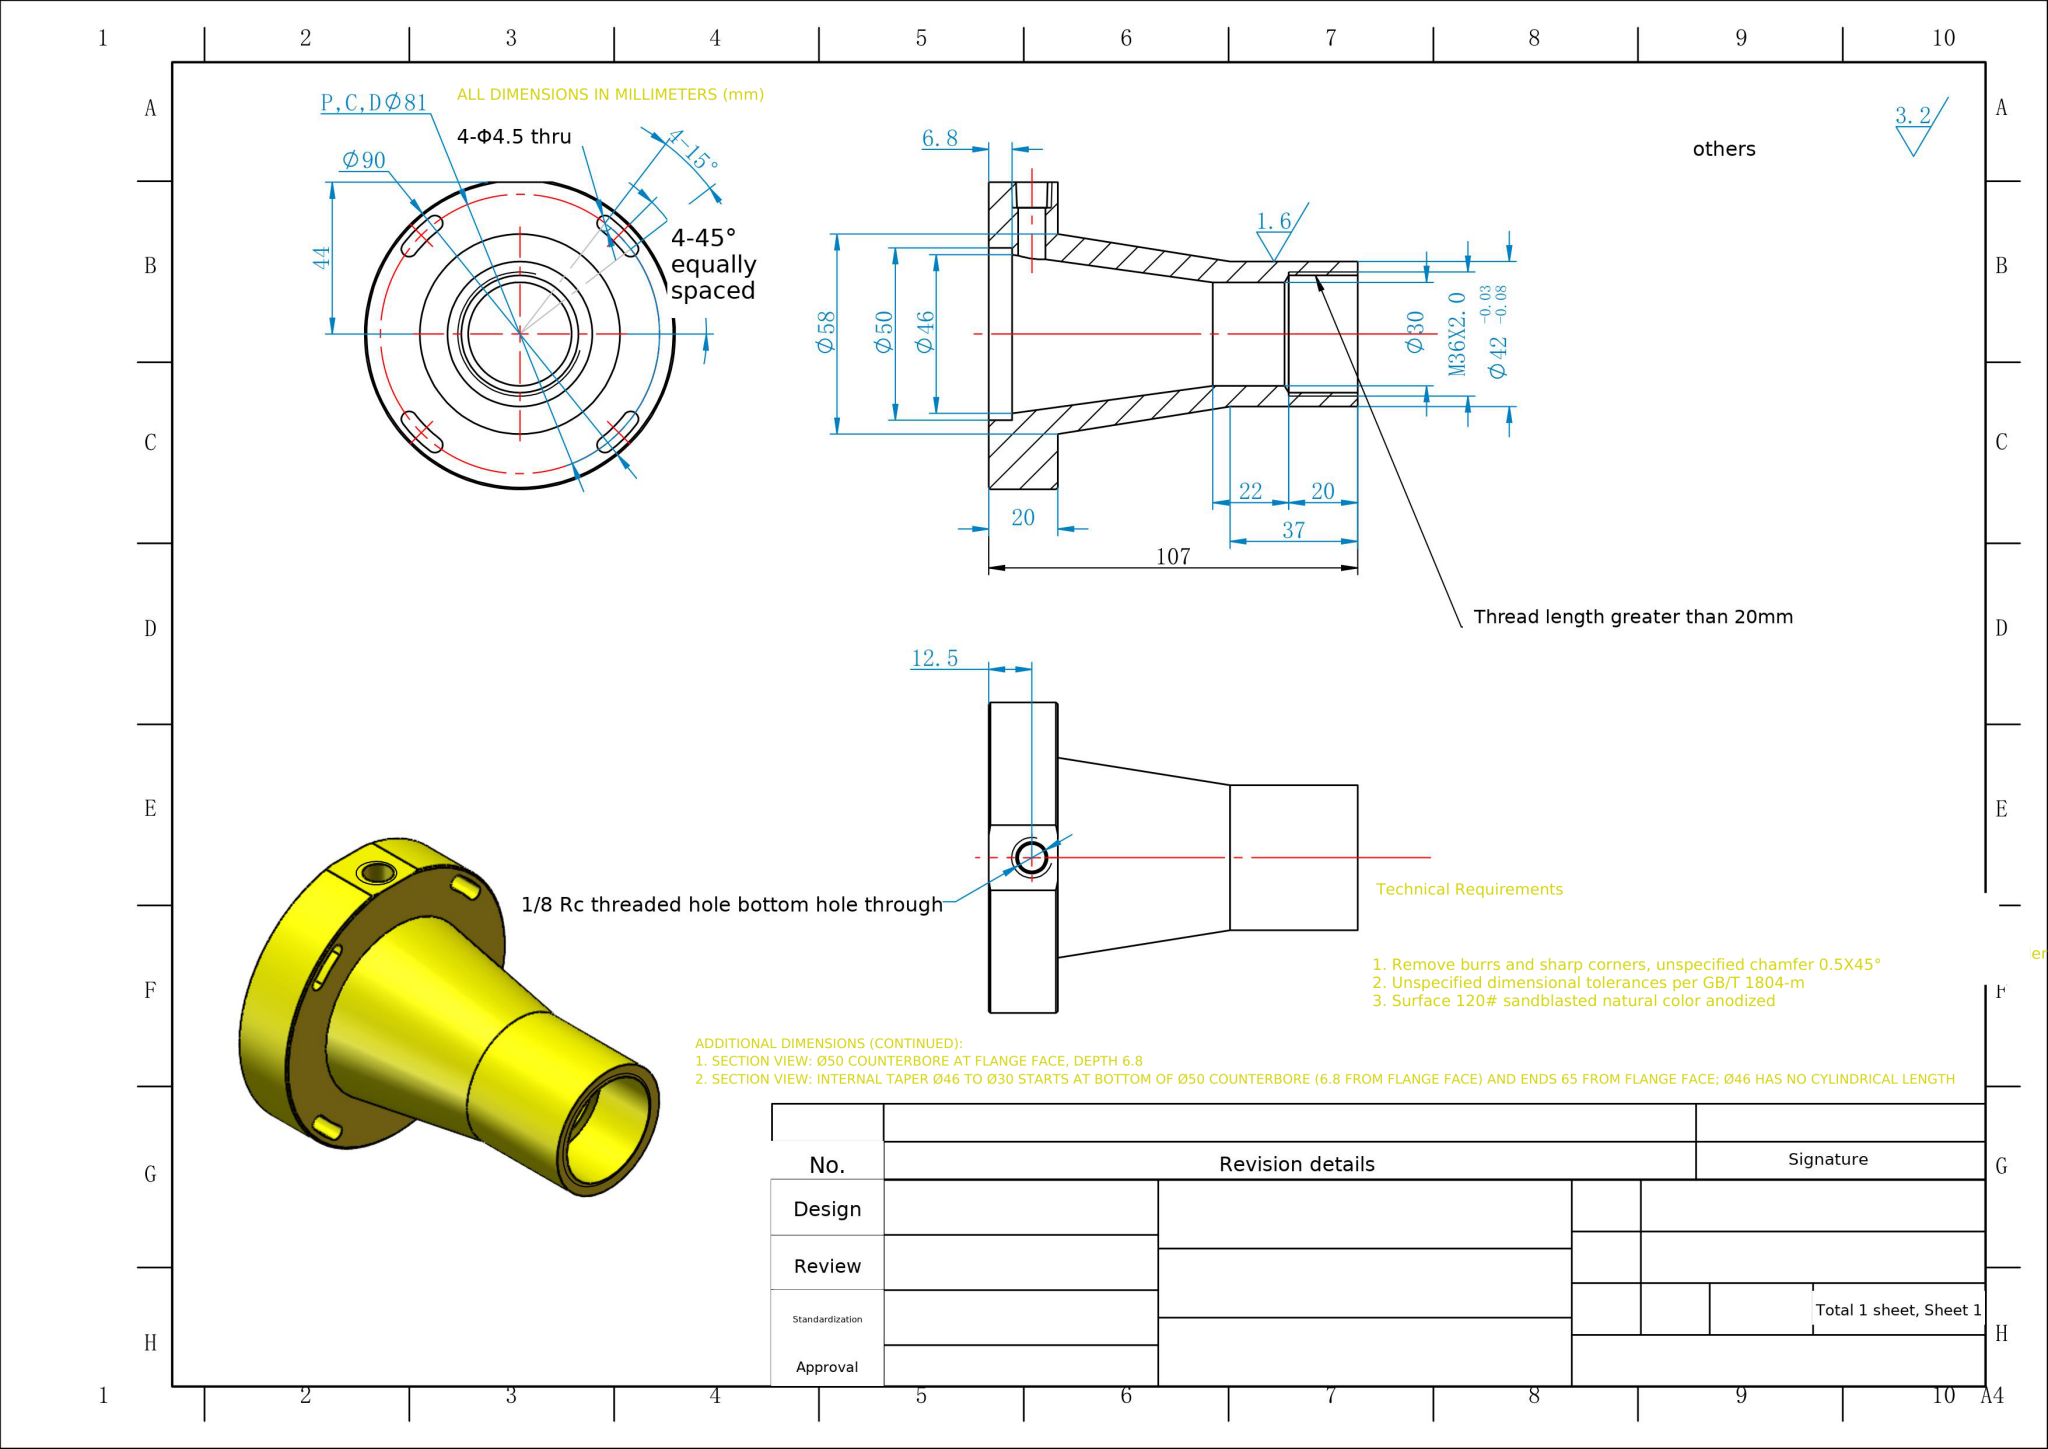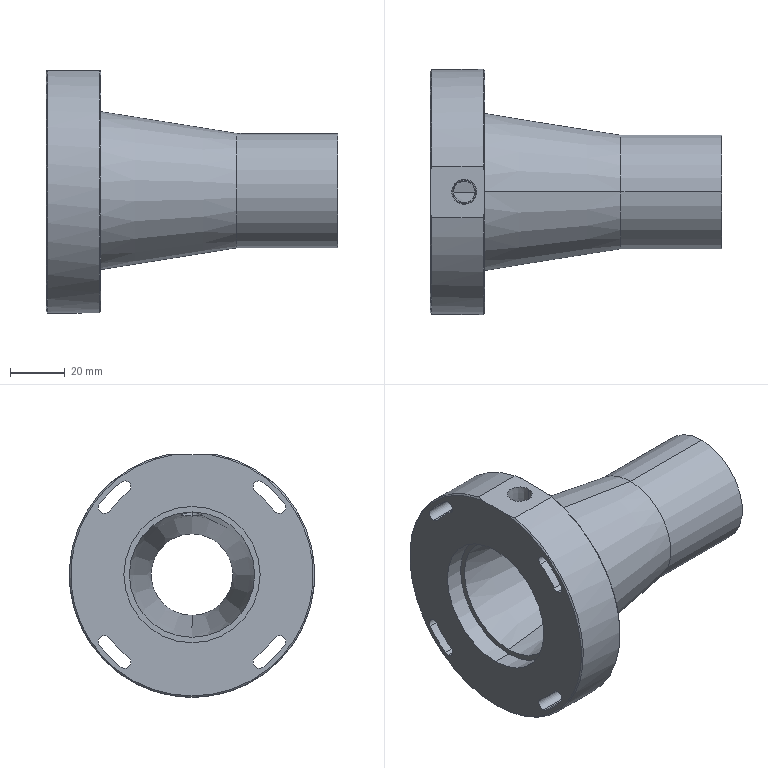Part | NX | mm | 1 solid | 48 faces | box 107 x 90 x 89 mm | volume 156769 mm3 | cylinder 31 | cone 11 | plane 6 | commonest cylinder face diameters 4.5 x12 76.5 x4 85.5 x4 34 x2 7.9 x2 30 x2 42 x2 50 x2